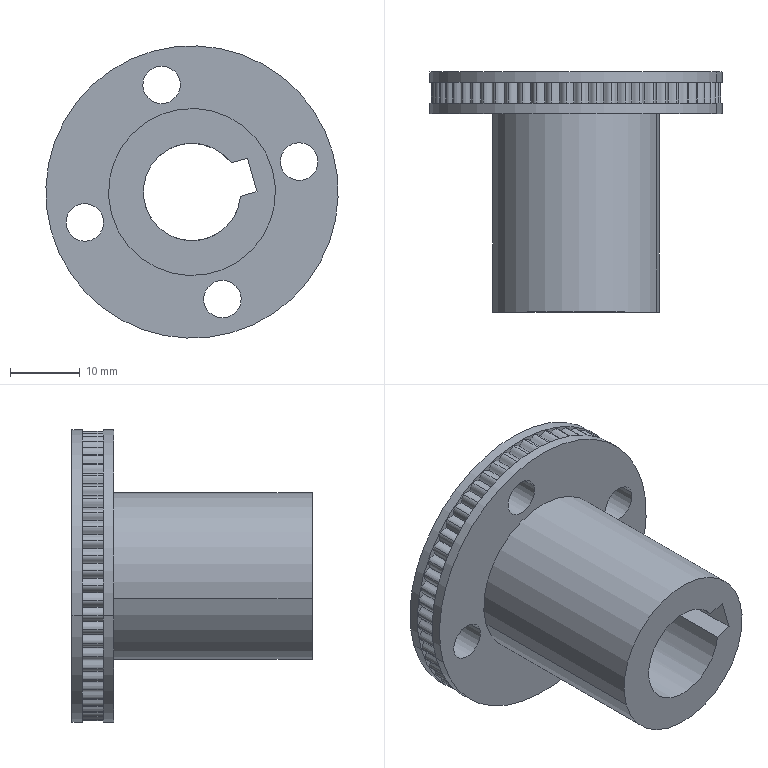Component | SolidWorks | DrivePart-1 | 1 solid | 143 faces | volume 14790 mm3 | spline 120 | cylinder 15 | plane 8 | commonest cylinder face diameters 5.4 x8 42 x4 24 x2 14 x1